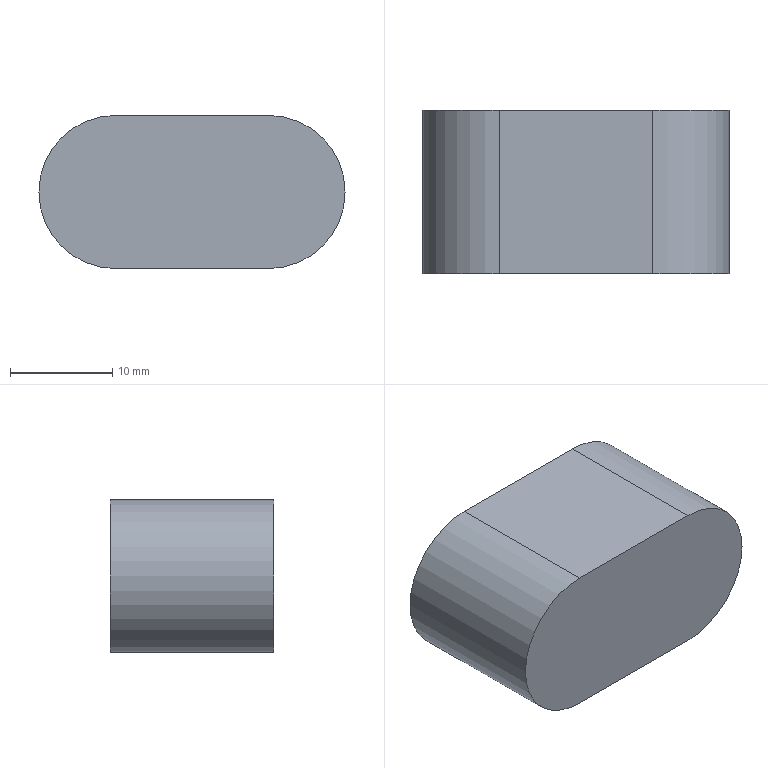Component | NX | PULLEY_KEY | 1 solid | 6 faces | box 30 x 16 x 15 mm | volume 6427 mm3 | plane 4 | cylinder 2 | commonest cylinder face diameters 15 x2
STEP:
#1=CARTESIAN_POINT('',(0.,0.,0.));
#2=DIRECTION('',(0.,0.,1.));
#3=DIRECTION('',(1.,0.,0.));
#4=AXIS2_PLACEMENT_3D('',#1,#2,#3);
#5=CARTESIAN_POINT('',(-133.042,-1160.882,832.497));
#6=VERTEX_POINT('',#5);
#7=CARTESIAN_POINT('',(-133.042,-1160.882,847.497));
#8=VERTEX_POINT('',#7);
#9=CARTESIAN_POINT('',(-133.042,-1160.882,839.997));
#10=DIRECTION('',(0.,1.,0.));
#11=DIRECTION('',(1.,0.,0.));
#12=AXIS2_PLACEMENT_3D('',#9,#10,#11);
#13=CIRCLE('',#12,7.5);
#14=CARTESIAN_POINT('',(-133.042,-1144.882,839.997));
#15=DIRECTION('',(0.,-1.,0.));
#16=DIRECTION('',(-1.,0.,0.));
#17=AXIS2_PLACEMENT_3D('',#14,#15,#16);
#18=CYLINDRICAL_SURFACE('',#17,7.5);
#19=CARTESIAN_POINT('',(3.142,16.));
#20=DIRECTION('',(-1.,0.));
#21=VECTOR('',#20,1.);
#22=LINE('',#19,#21);
#23=(GEOMETRIC_REPRESENTATION_CONTEXT(2)PARAMETRIC_REPRESENTATION_CONTEXT()REPRESENTATION_CONTEXT('',''));
#24=DEFINITIONAL_REPRESENTATION('',(#22),#23);
#25=PCURVE('',#18,#24);
#26=CARTESIAN_POINT('',(-133.042,-1160.882,839.997));
#27=DIRECTION('',(0.,1.,0.));
#28=DIRECTION('',(1.,0.,0.));
#29=AXIS2_PLACEMENT_3D('',#26,#27,#28);
#30=PLANE('',#29);
#31=CARTESIAN_POINT('',(0.,0.));
#32=DIRECTION('',(1.,0.));
#33=AXIS2_PLACEMENT_2D('',#31,#32);
#34=CIRCLE('',#33,7.5);
#35=(GEOMETRIC_REPRESENTATION_CONTEXT(2)PARAMETRIC_REPRESENTATION_CONTEXT()REPRESENTATION_CONTEXT('',''));
#36=DEFINITIONAL_REPRESENTATION('',(#34),#35);
#37=PCURVE('',#30,#36);
#38=SURFACE_CURVE('',#13,(#25,#37),.PCURVE_S1.);
#39=EDGE_CURVE('',#6,#8,#38,.T.);
#40=ORIENTED_EDGE('',*,*,#39,.T.);
#41=CARTESIAN_POINT('',(-133.042,-1144.882,847.497));
#42=VERTEX_POINT('',#41);
#43=CARTESIAN_POINT('',(-133.042,-1144.882,847.497));
#44=DIRECTION('',(0.,-1.,0.));
#45=VECTOR('',#44,1.);
#46=LINE('',#43,#45);
#47=CARTESIAN_POINT('',(-1.571,0.));
#48=DIRECTION('',(0.,1.));
#49=VECTOR('',#48,1.);
#50=LINE('',#47,#49);
#51=(GEOMETRIC_REPRESENTATION_CONTEXT(2)PARAMETRIC_REPRESENTATION_CONTEXT()REPRESENTATION_CONTEXT('',''));
#52=DEFINITIONAL_REPRESENTATION('',(#50),#51);
#53=PCURVE('',#18,#52);
#54=CARTESIAN_POINT('',(-133.042,-1144.882,847.497));
#55=DIRECTION('',(0.,0.,-1.));
#56=DIRECTION('',(0.,1.,0.));
#57=AXIS2_PLACEMENT_3D('',#54,#55,#56);
#58=PLANE('',#57);
#59=CARTESIAN_POINT('',(0.,0.));
#60=DIRECTION('',(-1.,0.));
#61=VECTOR('',#60,1.);
#62=LINE('',#59,#61);
#63=(GEOMETRIC_REPRESENTATION_CONTEXT(2)PARAMETRIC_REPRESENTATION_CONTEXT()REPRESENTATION_CONTEXT('',''));
#64=DEFINITIONAL_REPRESENTATION('',(#62),#63);
#65=PCURVE('',#58,#64);
#66=SURFACE_CURVE('',#46,(#53,#65),.PCURVE_S1.);
#67=EDGE_CURVE('',#42,#8,#66,.T.);
#68=ORIENTED_EDGE('',*,*,#67,.F.);
#69=CARTESIAN_POINT('',(-133.042,-1144.882,832.497));
#70=VERTEX_POINT('',#69);
#71=CARTESIAN_POINT('',(-133.042,-1144.882,839.997));
#72=DIRECTION('',(0.,1.,0.));
#73=DIRECTION('',(1.,0.,0.));
#74=AXIS2_PLACEMENT_3D('',#71,#72,#73);
#75=CIRCLE('',#74,7.5);
#76=CARTESIAN_POINT('',(3.142,0.));
#77=DIRECTION('',(-1.,0.));
#78=VECTOR('',#77,1.);
#79=LINE('',#76,#78);
#80=(GEOMETRIC_REPRESENTATION_CONTEXT(2)PARAMETRIC_REPRESENTATION_CONTEXT()REPRESENTATION_CONTEXT('',''));
#81=DEFINITIONAL_REPRESENTATION('',(#79),#80);
#82=PCURVE('',#18,#81);
#83=CARTESIAN_POINT('',(-133.042,-1144.882,839.997));
#84=DIRECTION('',(0.,1.,0.));
#85=DIRECTION('',(1.,0.,0.));
#86=AXIS2_PLACEMENT_3D('',#83,#84,#85);
#87=PLANE('',#86);
#88=CARTESIAN_POINT('',(0.,0.));
#89=DIRECTION('',(1.,0.));
#90=AXIS2_PLACEMENT_2D('',#88,#89);
#91=CIRCLE('',#90,7.5);
#92=(GEOMETRIC_REPRESENTATION_CONTEXT(2)PARAMETRIC_REPRESENTATION_CONTEXT()REPRESENTATION_CONTEXT('',''));
#93=DEFINITIONAL_REPRESENTATION('',(#91),#92);
#94=PCURVE('',#87,#93);
#95=SURFACE_CURVE('',#75,(#82,#94),.PCURVE_S1.);
#96=EDGE_CURVE('',#70,#42,#95,.T.);
#97=ORIENTED_EDGE('',*,*,#96,.F.);
#98=CARTESIAN_POINT('',(-133.042,-1144.882,832.497));
#99=DIRECTION('',(0.,-1.,0.));
#100=VECTOR('',#99,1.);
#101=LINE('',#98,#100);
#102=CARTESIAN_POINT('',(1.571,0.));
#103=DIRECTION('',(0.,1.));
#104=VECTOR('',#103,1.);
#105=LINE('',#102,#104);
#106=(GEOMETRIC_REPRESENTATION_CONTEXT(2)PARAMETRIC_REPRESENTATION_CONTEXT()REPRESENTATION_CONTEXT('',''));
#107=DEFINITIONAL_REPRESENTATION('',(#105),#106);
#108=PCURVE('',#18,#107);
#109=CARTESIAN_POINT('',(-118.042,-1144.882,832.497));
#110=DIRECTION('',(0.,0.,1.));
#111=DIRECTION('',(0.,-1.,0.));
#112=AXIS2_PLACEMENT_3D('',#109,#110,#111);
#113=PLANE('',#112);
#114=CARTESIAN_POINT('',(0.,-15.));
#115=DIRECTION('',(1.,0.));
#116=VECTOR('',#115,1.);
#117=LINE('',#114,#116);
#118=(GEOMETRIC_REPRESENTATION_CONTEXT(2)PARAMETRIC_REPRESENTATION_CONTEXT()REPRESENTATION_CONTEXT('',''));
#119=DEFINITIONAL_REPRESENTATION('',(#117),#118);
#120=PCURVE('',#113,#119);
#121=SURFACE_CURVE('',#101,(#108,#120),.PCURVE_S1.);
#122=EDGE_CURVE('',#70,#6,#121,.T.);
#123=ORIENTED_EDGE('',*,*,#122,.T.);
#124=EDGE_LOOP('',(#40,#68,#97,#123));
#125=FACE_BOUND('',#124,.T.);
#126=ADVANCED_FACE('',(#125),#18,.T.);
#127=CARTESIAN_POINT('',(-118.042,-1160.882,847.497));
#128=VERTEX_POINT('',#127);
#129=CARTESIAN_POINT('',(-133.042,-1160.882,847.497));
#130=DIRECTION('',(1.,0.,0.));
#131=VECTOR('',#130,1.);
#132=LINE('',#129,#131);
#133=CARTESIAN_POINT('',(-16.,0.));
#134=DIRECTION('',(0.,1.));
#135=VECTOR('',#134,1.);
#136=LINE('',#133,#135);
#137=(GEOMETRIC_REPRESENTATION_CONTEXT(2)PARAMETRIC_REPRESENTATION_CONTEXT()REPRESENTATION_CONTEXT('',''));
#138=DEFINITIONAL_REPRESENTATION('',(#136),#137);
#139=PCURVE('',#58,#138);
#140=CARTESIAN_POINT('',(0.,-7.5));
#141=DIRECTION('',(1.,0.));
#142=VECTOR('',#141,1.);
#143=LINE('',#140,#142);
#144=(GEOMETRIC_REPRESENTATION_CONTEXT(2)PARAMETRIC_REPRESENTATION_CONTEXT()REPRESENTATION_CONTEXT('',''));
#145=DEFINITIONAL_REPRESENTATION('',(#143),#144);
#146=PCURVE('',#30,#145);
#147=SURFACE_CURVE('',#132,(#139,#146),.PCURVE_S1.);
#148=EDGE_CURVE('',#8,#128,#147,.T.);
#149=ORIENTED_EDGE('',*,*,#148,.T.);
#150=CARTESIAN_POINT('',(-118.042,-1144.882,847.497));
#151=VERTEX_POINT('',#150);
#152=CARTESIAN_POINT('',(-118.042,-1144.882,847.497));
#153=DIRECTION('',(0.,-1.,0.));
#154=VECTOR('',#153,1.);
#155=LINE('',#152,#154);
#156=CARTESIAN_POINT('',(0.,15.));
#157=DIRECTION('',(-1.,0.));
#158=VECTOR('',#157,1.);
#159=LINE('',#156,#158);
#160=(GEOMETRIC_REPRESENTATION_CONTEXT(2)PARAMETRIC_REPRESENTATION_CONTEXT()REPRESENTATION_CONTEXT('',''));
#161=DEFINITIONAL_REPRESENTATION('',(#159),#160);
#162=PCURVE('',#58,#161);
#163=CARTESIAN_POINT('',(-118.042,-1144.882,839.997));
#164=DIRECTION('',(0.,-1.,0.));
#165=DIRECTION('',(-1.,0.,0.));
#166=AXIS2_PLACEMENT_3D('',#163,#164,#165);
#167=CYLINDRICAL_SURFACE('',#166,7.5);
#168=CARTESIAN_POINT('',(4.712,0.));
#169=DIRECTION('',(0.,1.));
#170=VECTOR('',#169,1.);
#171=LINE('',#168,#170);
#172=(GEOMETRIC_REPRESENTATION_CONTEXT(2)PARAMETRIC_REPRESENTATION_CONTEXT()REPRESENTATION_CONTEXT('',''));
#173=DEFINITIONAL_REPRESENTATION('',(#171),#172);
#174=PCURVE('',#167,#173);
#175=SURFACE_CURVE('',#155,(#162,#174),.PCURVE_S1.);
#176=EDGE_CURVE('',#151,#128,#175,.T.);
#177=ORIENTED_EDGE('',*,*,#176,.F.);
#178=CARTESIAN_POINT('',(-133.042,-1144.882,847.497));
#179=DIRECTION('',(1.,0.,0.));
#180=VECTOR('',#179,1.);
#181=LINE('',#178,#180);
#182=CARTESIAN_POINT('',(0.,0.));
#183=DIRECTION('',(0.,1.));
#184=VECTOR('',#183,1.);
#185=LINE('',#182,#184);
#186=(GEOMETRIC_REPRESENTATION_CONTEXT(2)PARAMETRIC_REPRESENTATION_CONTEXT()REPRESENTATION_CONTEXT('',''));
#187=DEFINITIONAL_REPRESENTATION('',(#185),#186);
#188=PCURVE('',#58,#187);
#189=CARTESIAN_POINT('',(0.,-7.5));
#190=DIRECTION('',(1.,0.));
#191=VECTOR('',#190,1.);
#192=LINE('',#189,#191);
#193=(GEOMETRIC_REPRESENTATION_CONTEXT(2)PARAMETRIC_REPRESENTATION_CONTEXT()REPRESENTATION_CONTEXT('',''));
#194=DEFINITIONAL_REPRESENTATION('',(#192),#193);
#195=PCURVE('',#87,#194);
#196=SURFACE_CURVE('',#181,(#188,#195),.PCURVE_S1.);
#197=EDGE_CURVE('',#42,#151,#196,.T.);
#198=ORIENTED_EDGE('',*,*,#197,.F.);
#199=ORIENTED_EDGE('',*,*,#67,.T.);
#200=EDGE_LOOP('',(#149,#177,#198,#199));
#201=FACE_BOUND('',#200,.T.);
#202=ADVANCED_FACE('',(#201),#58,.F.);
#203=CARTESIAN_POINT('',(-118.042,-1160.882,832.497));
#204=VERTEX_POINT('',#203);
#205=CARTESIAN_POINT('',(-118.042,-1160.882,839.997));
#206=DIRECTION('',(0.,1.,0.));
#207=DIRECTION('',(1.,0.,0.));
#208=AXIS2_PLACEMENT_3D('',#205,#206,#207);
#209=CIRCLE('',#208,7.5);
#210=CARTESIAN_POINT('',(9.425,16.));
#211=DIRECTION('',(-1.,0.));
#212=VECTOR('',#211,1.);
#213=LINE('',#210,#212);
#214=(GEOMETRIC_REPRESENTATION_CONTEXT(2)PARAMETRIC_REPRESENTATION_CONTEXT()REPRESENTATION_CONTEXT('',''));
#215=DEFINITIONAL_REPRESENTATION('',(#213),#214);
#216=PCURVE('',#167,#215);
#217=CARTESIAN_POINT('',(15.,0.));
#218=DIRECTION('',(1.,0.));
#219=AXIS2_PLACEMENT_2D('',#217,#218);
#220=CIRCLE('',#219,7.5);
#221=(GEOMETRIC_REPRESENTATION_CONTEXT(2)PARAMETRIC_REPRESENTATION_CONTEXT()REPRESENTATION_CONTEXT('',''));
#222=DEFINITIONAL_REPRESENTATION('',(#220),#221);
#223=PCURVE('',#30,#222);
#224=SURFACE_CURVE('',#209,(#216,#223),.PCURVE_S1.);
#225=EDGE_CURVE('',#128,#204,#224,.T.);
#226=ORIENTED_EDGE('',*,*,#225,.T.);
#227=CARTESIAN_POINT('',(-118.042,-1144.882,832.497));
#228=VERTEX_POINT('',#227);
#229=CARTESIAN_POINT('',(-118.042,-1144.882,832.497));
#230=DIRECTION('',(0.,-1.,0.));
#231=VECTOR('',#230,1.);
#232=LINE('',#229,#231);
#233=CARTESIAN_POINT('',(1.571,0.));
#234=DIRECTION('',(0.,1.));
#235=VECTOR('',#234,1.);
#236=LINE('',#233,#235);
#237=(GEOMETRIC_REPRESENTATION_CONTEXT(2)PARAMETRIC_REPRESENTATION_CONTEXT()REPRESENTATION_CONTEXT('',''));
#238=DEFINITIONAL_REPRESENTATION('',(#236),#237);
#239=PCURVE('',#167,#238);
#240=CARTESIAN_POINT('',(0.,0.));
#241=DIRECTION('',(1.,0.));
#242=VECTOR('',#241,1.);
#243=LINE('',#240,#242);
#244=(GEOMETRIC_REPRESENTATION_CONTEXT(2)PARAMETRIC_REPRESENTATION_CONTEXT()REPRESENTATION_CONTEXT('',''));
#245=DEFINITIONAL_REPRESENTATION('',(#243),#244);
#246=PCURVE('',#113,#245);
#247=SURFACE_CURVE('',#232,(#239,#246),.PCURVE_S1.);
#248=EDGE_CURVE('',#228,#204,#247,.T.);
#249=ORIENTED_EDGE('',*,*,#248,.F.);
#250=CARTESIAN_POINT('',(-118.042,-1144.882,839.997));
#251=DIRECTION('',(0.,1.,0.));
#252=DIRECTION('',(1.,0.,0.));
#253=AXIS2_PLACEMENT_3D('',#250,#251,#252);
#254=CIRCLE('',#253,7.5);
#255=CARTESIAN_POINT('',(9.425,0.));
#256=DIRECTION('',(-1.,0.));
#257=VECTOR('',#256,1.);
#258=LINE('',#255,#257);
#259=(GEOMETRIC_REPRESENTATION_CONTEXT(2)PARAMETRIC_REPRESENTATION_CONTEXT()REPRESENTATION_CONTEXT('',''));
#260=DEFINITIONAL_REPRESENTATION('',(#258),#259);
#261=PCURVE('',#167,#260);
#262=CARTESIAN_POINT('',(15.,0.));
#263=DIRECTION('',(1.,0.));
#264=AXIS2_PLACEMENT_2D('',#262,#263);
#265=CIRCLE('',#264,7.5);
#266=(GEOMETRIC_REPRESENTATION_CONTEXT(2)PARAMETRIC_REPRESENTATION_CONTEXT()REPRESENTATION_CONTEXT('',''));
#267=DEFINITIONAL_REPRESENTATION('',(#265),#266);
#268=PCURVE('',#87,#267);
#269=SURFACE_CURVE('',#254,(#261,#268),.PCURVE_S1.);
#270=EDGE_CURVE('',#151,#228,#269,.T.);
#271=ORIENTED_EDGE('',*,*,#270,.F.);
#272=ORIENTED_EDGE('',*,*,#176,.T.);
#273=EDGE_LOOP('',(#226,#249,#271,#272));
#274=FACE_BOUND('',#273,.T.);
#275=ADVANCED_FACE('',(#274),#167,.T.);
#276=CARTESIAN_POINT('',(-118.042,-1160.882,832.497));
#277=DIRECTION('',(-1.,0.,0.));
#278=VECTOR('',#277,1.);
#279=LINE('',#276,#278);
#280=CARTESIAN_POINT('',(16.,0.));
#281=DIRECTION('',(0.,-1.));
#282=VECTOR('',#281,1.);
#283=LINE('',#280,#282);
#284=(GEOMETRIC_REPRESENTATION_CONTEXT(2)PARAMETRIC_REPRESENTATION_CONTEXT()REPRESENTATION_CONTEXT('',''));
#285=DEFINITIONAL_REPRESENTATION('',(#283),#284);
#286=PCURVE('',#113,#285);
#287=CARTESIAN_POINT('',(15.,7.5));
#288=DIRECTION('',(-1.,0.));
#289=VECTOR('',#288,1.);
#290=LINE('',#287,#289);
#291=(GEOMETRIC_REPRESENTATION_CONTEXT(2)PARAMETRIC_REPRESENTATION_CONTEXT()REPRESENTATION_CONTEXT('',''));
#292=DEFINITIONAL_REPRESENTATION('',(#290),#291);
#293=PCURVE('',#30,#292);
#294=SURFACE_CURVE('',#279,(#286,#293),.PCURVE_S1.);
#295=EDGE_CURVE('',#204,#6,#294,.T.);
#296=ORIENTED_EDGE('',*,*,#295,.T.);
#297=ORIENTED_EDGE('',*,*,#122,.F.);
#298=CARTESIAN_POINT('',(-118.042,-1144.882,832.497));
#299=DIRECTION('',(-1.,0.,0.));
#300=VECTOR('',#299,1.);
#301=LINE('',#298,#300);
#302=CARTESIAN_POINT('',(0.,0.));
#303=DIRECTION('',(0.,-1.));
#304=VECTOR('',#303,1.);
#305=LINE('',#302,#304);
#306=(GEOMETRIC_REPRESENTATION_CONTEXT(2)PARAMETRIC_REPRESENTATION_CONTEXT()REPRESENTATION_CONTEXT('',''));
#307=DEFINITIONAL_REPRESENTATION('',(#305),#306);
#308=PCURVE('',#113,#307);
#309=CARTESIAN_POINT('',(15.,7.5));
#310=DIRECTION('',(-1.,0.));
#311=VECTOR('',#310,1.);
#312=LINE('',#309,#311);
#313=(GEOMETRIC_REPRESENTATION_CONTEXT(2)PARAMETRIC_REPRESENTATION_CONTEXT()REPRESENTATION_CONTEXT('',''));
#314=DEFINITIONAL_REPRESENTATION('',(#312),#313);
#315=PCURVE('',#87,#314);
#316=SURFACE_CURVE('',#301,(#308,#315),.PCURVE_S1.);
#317=EDGE_CURVE('',#228,#70,#316,.T.);
#318=ORIENTED_EDGE('',*,*,#317,.F.);
#319=ORIENTED_EDGE('',*,*,#248,.T.);
#320=EDGE_LOOP('',(#296,#297,#318,#319));
#321=FACE_BOUND('',#320,.T.);
#322=ADVANCED_FACE('',(#321),#113,.F.);
#323=ORIENTED_EDGE('',*,*,#96,.T.);
#324=ORIENTED_EDGE('',*,*,#197,.T.);
#325=ORIENTED_EDGE('',*,*,#270,.T.);
#326=ORIENTED_EDGE('',*,*,#317,.T.);
#327=EDGE_LOOP('',(#323,#324,#325,#326));
#328=FACE_BOUND('',#327,.T.);
#329=ADVANCED_FACE('',(#328),#87,.T.);
#330=ORIENTED_EDGE('',*,*,#39,.F.);
#331=ORIENTED_EDGE('',*,*,#295,.F.);
#332=ORIENTED_EDGE('',*,*,#225,.F.);
#333=ORIENTED_EDGE('',*,*,#148,.F.);
#334=EDGE_LOOP('',(#330,#331,#332,#333));
#335=FACE_BOUND('',#334,.T.);
#336=ADVANCED_FACE('',(#335),#30,.F.);
#337=CLOSED_SHELL('',(#126,#202,#275,#322,#329,#336));
#338=MANIFOLD_SOLID_BREP('',#337);
#339=(LENGTH_UNIT()NAMED_UNIT(*)SI_UNIT(.MILLI.,.METRE.));
#340=UNCERTAINTY_MEASURE_WITH_UNIT(LENGTH_MEASURE(0.0000001),#339,'','');
#341=(NAMED_UNIT(*)PLANE_ANGLE_UNIT()SI_UNIT($,.RADIAN.));
#342=(NAMED_UNIT(*)SI_UNIT($,.STERADIAN.)SOLID_ANGLE_UNIT());
#343=(GEOMETRIC_REPRESENTATION_CONTEXT(3)GLOBAL_UNCERTAINTY_ASSIGNED_CONTEXT((#340))GLOBAL_UNIT_ASSIGNED_CONTEXT((#339,#341,#342))REPRESENTATION_CONTEXT('',''));
#344=ADVANCED_BREP_SHAPE_REPRESENTATION('',(#4,#338),#343);